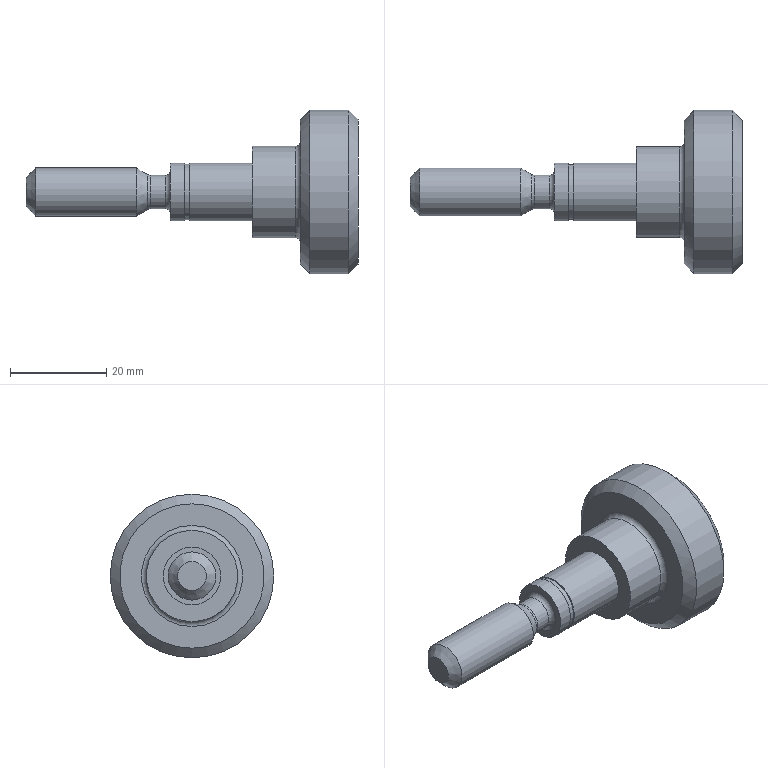Component | NX | LEADSCREW | 1 solid | 21 faces | volume 17319 mm3 | plane 7 | cylinder 7 | cone 4 | torus 3 | commonest cylinder face diameters 12 x2 34 x1 19 x1 11.5 x1 7 x1 10 x1